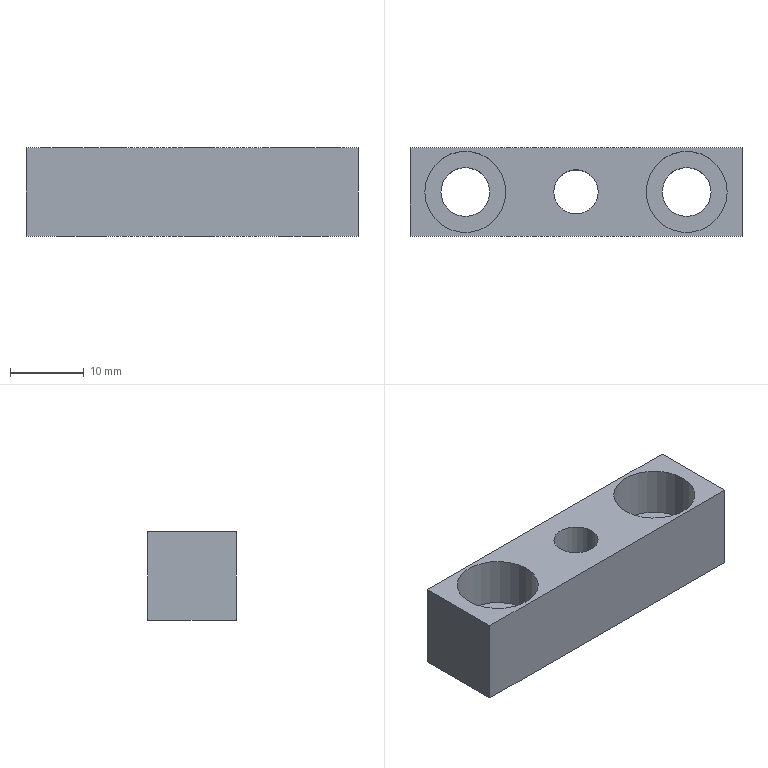Component | NX | GUIDE_BLOCK | 1 solid | 13 faces | box 45 x 12 x 12 mm | volume 4492 mm3 | plane 8 | cylinder 5 | commonest cylinder face diameters 6.6 x2 11 x2 6 x1
STEP:
#1=CARTESIAN_POINT('',(0.,0.,0.));
#2=DIRECTION('',(0.,0.,1.));
#3=DIRECTION('',(1.,0.,0.));
#4=AXIS2_PLACEMENT_3D('',#1,#2,#3);
#5=CARTESIAN_POINT('',(-95.,33.,10.));
#6=VERTEX_POINT('',#5);
#7=CARTESIAN_POINT('',(-95.,21.,10.));
#8=VERTEX_POINT('',#7);
#9=CARTESIAN_POINT('',(-95.,33.,10.));
#10=DIRECTION('',(0.,-1.,0.));
#11=VECTOR('',#10,1.);
#12=LINE('',#9,#11);
#13=CARTESIAN_POINT('',(-95.,33.,22.));
#14=DIRECTION('',(1.,0.,0.));
#15=DIRECTION('',(0.,0.,-1.));
#16=AXIS2_PLACEMENT_3D('',#13,#14,#15);
#17=PLANE('',#16);
#18=CARTESIAN_POINT('',(12.,0.));
#19=DIRECTION('',(0.,-1.));
#20=VECTOR('',#19,1.);
#21=LINE('',#18,#20);
#22=(GEOMETRIC_REPRESENTATION_CONTEXT(2)PARAMETRIC_REPRESENTATION_CONTEXT()REPRESENTATION_CONTEXT('',''));
#23=DEFINITIONAL_REPRESENTATION('',(#21),#22);
#24=PCURVE('',#17,#23);
#25=CARTESIAN_POINT('',(-72.5,27.,10.));
#26=DIRECTION('',(0.,0.,1.));
#27=DIRECTION('',(1.,0.,0.));
#28=AXIS2_PLACEMENT_3D('',#25,#26,#27);
#29=PLANE('',#28);
#30=CARTESIAN_POINT('',(-22.5,6.));
#31=DIRECTION('',(0.,-1.));
#32=VECTOR('',#31,1.);
#33=LINE('',#30,#32);
#34=(GEOMETRIC_REPRESENTATION_CONTEXT(2)PARAMETRIC_REPRESENTATION_CONTEXT()REPRESENTATION_CONTEXT('',''));
#35=DEFINITIONAL_REPRESENTATION('',(#33),#34);
#36=PCURVE('',#29,#35);
#37=SURFACE_CURVE('',#12,(#24,#36),.PCURVE_S1.);
#38=EDGE_CURVE('',#6,#8,#37,.T.);
#39=ORIENTED_EDGE('',*,*,#38,.T.);
#40=CARTESIAN_POINT('',(-95.,21.,22.));
#41=VERTEX_POINT('',#40);
#42=CARTESIAN_POINT('',(-95.,21.,22.));
#43=DIRECTION('',(0.,0.,-1.));
#44=VECTOR('',#43,1.);
#45=LINE('',#42,#44);
#46=CARTESIAN_POINT('',(0.,-12.));
#47=DIRECTION('',(1.,0.));
#48=VECTOR('',#47,1.);
#49=LINE('',#46,#48);
#50=(GEOMETRIC_REPRESENTATION_CONTEXT(2)PARAMETRIC_REPRESENTATION_CONTEXT()REPRESENTATION_CONTEXT('',''));
#51=DEFINITIONAL_REPRESENTATION('',(#49),#50);
#52=PCURVE('',#17,#51);
#53=CARTESIAN_POINT('',(-95.,21.,22.));
#54=DIRECTION('',(0.,1.,0.));
#55=DIRECTION('',(0.,0.,1.));
#56=AXIS2_PLACEMENT_3D('',#53,#54,#55);
#57=PLANE('',#56);
#58=CARTESIAN_POINT('',(0.,0.));
#59=DIRECTION('',(-1.,0.));
#60=VECTOR('',#59,1.);
#61=LINE('',#58,#60);
#62=(GEOMETRIC_REPRESENTATION_CONTEXT(2)PARAMETRIC_REPRESENTATION_CONTEXT()REPRESENTATION_CONTEXT('',''));
#63=DEFINITIONAL_REPRESENTATION('',(#61),#62);
#64=PCURVE('',#57,#63);
#65=SURFACE_CURVE('',#45,(#52,#64),.PCURVE_S1.);
#66=EDGE_CURVE('',#41,#8,#65,.T.);
#67=ORIENTED_EDGE('',*,*,#66,.F.);
#68=CARTESIAN_POINT('',(-95.,33.,22.));
#69=VERTEX_POINT('',#68);
#70=CARTESIAN_POINT('',(-95.,33.,22.));
#71=DIRECTION('',(0.,-1.,0.));
#72=VECTOR('',#71,1.);
#73=LINE('',#70,#72);
#74=CARTESIAN_POINT('',(0.,0.));
#75=DIRECTION('',(0.,-1.));
#76=VECTOR('',#75,1.);
#77=LINE('',#74,#76);
#78=(GEOMETRIC_REPRESENTATION_CONTEXT(2)PARAMETRIC_REPRESENTATION_CONTEXT()REPRESENTATION_CONTEXT('',''));
#79=DEFINITIONAL_REPRESENTATION('',(#77),#78);
#80=PCURVE('',#17,#79);
#81=CARTESIAN_POINT('',(-72.5,27.,22.));
#82=DIRECTION('',(0.,0.,1.));
#83=DIRECTION('',(1.,0.,0.));
#84=AXIS2_PLACEMENT_3D('',#81,#82,#83);
#85=PLANE('',#84);
#86=CARTESIAN_POINT('',(-22.5,6.));
#87=DIRECTION('',(0.,-1.));
#88=VECTOR('',#87,1.);
#89=LINE('',#86,#88);
#90=(GEOMETRIC_REPRESENTATION_CONTEXT(2)PARAMETRIC_REPRESENTATION_CONTEXT()REPRESENTATION_CONTEXT('',''));
#91=DEFINITIONAL_REPRESENTATION('',(#89),#90);
#92=PCURVE('',#85,#91);
#93=SURFACE_CURVE('',#73,(#80,#92),.PCURVE_S1.);
#94=EDGE_CURVE('',#69,#41,#93,.T.);
#95=ORIENTED_EDGE('',*,*,#94,.F.);
#96=CARTESIAN_POINT('',(-95.,33.,22.));
#97=DIRECTION('',(0.,0.,-1.));
#98=VECTOR('',#97,1.);
#99=LINE('',#96,#98);
#100=CARTESIAN_POINT('',(0.,0.));
#101=DIRECTION('',(1.,0.));
#102=VECTOR('',#101,1.);
#103=LINE('',#100,#102);
#104=(GEOMETRIC_REPRESENTATION_CONTEXT(2)PARAMETRIC_REPRESENTATION_CONTEXT()REPRESENTATION_CONTEXT('',''));
#105=DEFINITIONAL_REPRESENTATION('',(#103),#104);
#106=PCURVE('',#17,#105);
#107=CARTESIAN_POINT('',(-50.,33.,22.));
#108=DIRECTION('',(0.,-1.,0.));
#109=DIRECTION('',(0.,0.,-1.));
#110=AXIS2_PLACEMENT_3D('',#107,#108,#109);
#111=PLANE('',#110);
#112=CARTESIAN_POINT('',(0.,-45.));
#113=DIRECTION('',(1.,0.));
#114=VECTOR('',#113,1.);
#115=LINE('',#112,#114);
#116=(GEOMETRIC_REPRESENTATION_CONTEXT(2)PARAMETRIC_REPRESENTATION_CONTEXT()REPRESENTATION_CONTEXT('',''));
#117=DEFINITIONAL_REPRESENTATION('',(#115),#116);
#118=PCURVE('',#111,#117);
#119=SURFACE_CURVE('',#99,(#106,#118),.PCURVE_S1.);
#120=EDGE_CURVE('',#69,#6,#119,.T.);
#121=ORIENTED_EDGE('',*,*,#120,.T.);
#122=EDGE_LOOP('',(#39,#67,#95,#121));
#123=FACE_BOUND('',#122,.T.);
#124=ADVANCED_FACE('',(#123),#17,.F.);
#125=CARTESIAN_POINT('',(-50.,21.,10.));
#126=VERTEX_POINT('',#125);
#127=CARTESIAN_POINT('',(-95.,21.,10.));
#128=DIRECTION('',(1.,0.,0.));
#129=VECTOR('',#128,1.);
#130=LINE('',#127,#129);
#131=CARTESIAN_POINT('',(-12.,0.));
#132=DIRECTION('',(0.,1.));
#133=VECTOR('',#132,1.);
#134=LINE('',#131,#133);
#135=(GEOMETRIC_REPRESENTATION_CONTEXT(2)PARAMETRIC_REPRESENTATION_CONTEXT()REPRESENTATION_CONTEXT('',''));
#136=DEFINITIONAL_REPRESENTATION('',(#134),#135);
#137=PCURVE('',#57,#136);
#138=CARTESIAN_POINT('',(-22.5,-6.));
#139=DIRECTION('',(1.,0.));
#140=VECTOR('',#139,1.);
#141=LINE('',#138,#140);
#142=(GEOMETRIC_REPRESENTATION_CONTEXT(2)PARAMETRIC_REPRESENTATION_CONTEXT()REPRESENTATION_CONTEXT('',''));
#143=DEFINITIONAL_REPRESENTATION('',(#141),#142);
#144=PCURVE('',#29,#143);
#145=SURFACE_CURVE('',#130,(#137,#144),.PCURVE_S1.);
#146=EDGE_CURVE('',#8,#126,#145,.T.);
#147=ORIENTED_EDGE('',*,*,#146,.T.);
#148=CARTESIAN_POINT('',(-50.,21.,22.));
#149=VERTEX_POINT('',#148);
#150=CARTESIAN_POINT('',(-50.,21.,22.));
#151=DIRECTION('',(0.,0.,-1.));
#152=VECTOR('',#151,1.);
#153=LINE('',#150,#152);
#154=CARTESIAN_POINT('',(0.,45.));
#155=DIRECTION('',(-1.,0.));
#156=VECTOR('',#155,1.);
#157=LINE('',#154,#156);
#158=(GEOMETRIC_REPRESENTATION_CONTEXT(2)PARAMETRIC_REPRESENTATION_CONTEXT()REPRESENTATION_CONTEXT('',''));
#159=DEFINITIONAL_REPRESENTATION('',(#157),#158);
#160=PCURVE('',#57,#159);
#161=CARTESIAN_POINT('',(-50.,21.,22.));
#162=DIRECTION('',(-1.,0.,0.));
#163=DIRECTION('',(0.,0.,1.));
#164=AXIS2_PLACEMENT_3D('',#161,#162,#163);
#165=PLANE('',#164);
#166=CARTESIAN_POINT('',(0.,0.));
#167=DIRECTION('',(-1.,0.));
#168=VECTOR('',#167,1.);
#169=LINE('',#166,#168);
#170=(GEOMETRIC_REPRESENTATION_CONTEXT(2)PARAMETRIC_REPRESENTATION_CONTEXT()REPRESENTATION_CONTEXT('',''));
#171=DEFINITIONAL_REPRESENTATION('',(#169),#170);
#172=PCURVE('',#165,#171);
#173=SURFACE_CURVE('',#153,(#160,#172),.PCURVE_S1.);
#174=EDGE_CURVE('',#149,#126,#173,.T.);
#175=ORIENTED_EDGE('',*,*,#174,.F.);
#176=CARTESIAN_POINT('',(-95.,21.,22.));
#177=DIRECTION('',(1.,0.,0.));
#178=VECTOR('',#177,1.);
#179=LINE('',#176,#178);
#180=CARTESIAN_POINT('',(0.,0.));
#181=DIRECTION('',(0.,1.));
#182=VECTOR('',#181,1.);
#183=LINE('',#180,#182);
#184=(GEOMETRIC_REPRESENTATION_CONTEXT(2)PARAMETRIC_REPRESENTATION_CONTEXT()REPRESENTATION_CONTEXT('',''));
#185=DEFINITIONAL_REPRESENTATION('',(#183),#184);
#186=PCURVE('',#57,#185);
#187=CARTESIAN_POINT('',(-22.5,-6.));
#188=DIRECTION('',(1.,0.));
#189=VECTOR('',#188,1.);
#190=LINE('',#187,#189);
#191=(GEOMETRIC_REPRESENTATION_CONTEXT(2)PARAMETRIC_REPRESENTATION_CONTEXT()REPRESENTATION_CONTEXT('',''));
#192=DEFINITIONAL_REPRESENTATION('',(#190),#191);
#193=PCURVE('',#85,#192);
#194=SURFACE_CURVE('',#179,(#186,#193),.PCURVE_S1.);
#195=EDGE_CURVE('',#41,#149,#194,.T.);
#196=ORIENTED_EDGE('',*,*,#195,.F.);
#197=ORIENTED_EDGE('',*,*,#66,.T.);
#198=EDGE_LOOP('',(#147,#175,#196,#197));
#199=FACE_BOUND('',#198,.T.);
#200=ADVANCED_FACE('',(#199),#57,.F.);
#201=CARTESIAN_POINT('',(-50.,33.,10.));
#202=VERTEX_POINT('',#201);
#203=CARTESIAN_POINT('',(-50.,21.,10.));
#204=DIRECTION('',(0.,1.,0.));
#205=VECTOR('',#204,1.);
#206=LINE('',#203,#205);
#207=CARTESIAN_POINT('',(-12.,0.));
#208=DIRECTION('',(0.,1.));
#209=VECTOR('',#208,1.);
#210=LINE('',#207,#209);
#211=(GEOMETRIC_REPRESENTATION_CONTEXT(2)PARAMETRIC_REPRESENTATION_CONTEXT()REPRESENTATION_CONTEXT('',''));
#212=DEFINITIONAL_REPRESENTATION('',(#210),#211);
#213=PCURVE('',#165,#212);
#214=CARTESIAN_POINT('',(22.5,-6.));
#215=DIRECTION('',(0.,1.));
#216=VECTOR('',#215,1.);
#217=LINE('',#214,#216);
#218=(GEOMETRIC_REPRESENTATION_CONTEXT(2)PARAMETRIC_REPRESENTATION_CONTEXT()REPRESENTATION_CONTEXT('',''));
#219=DEFINITIONAL_REPRESENTATION('',(#217),#218);
#220=PCURVE('',#29,#219);
#221=SURFACE_CURVE('',#206,(#213,#220),.PCURVE_S1.);
#222=EDGE_CURVE('',#126,#202,#221,.T.);
#223=ORIENTED_EDGE('',*,*,#222,.T.);
#224=CARTESIAN_POINT('',(-50.,33.,22.));
#225=VERTEX_POINT('',#224);
#226=CARTESIAN_POINT('',(-50.,33.,22.));
#227=DIRECTION('',(0.,0.,-1.));
#228=VECTOR('',#227,1.);
#229=LINE('',#226,#228);
#230=CARTESIAN_POINT('',(0.,12.));
#231=DIRECTION('',(-1.,0.));
#232=VECTOR('',#231,1.);
#233=LINE('',#230,#232);
#234=(GEOMETRIC_REPRESENTATION_CONTEXT(2)PARAMETRIC_REPRESENTATION_CONTEXT()REPRESENTATION_CONTEXT('',''));
#235=DEFINITIONAL_REPRESENTATION('',(#233),#234);
#236=PCURVE('',#165,#235);
#237=CARTESIAN_POINT('',(0.,0.));
#238=DIRECTION('',(1.,0.));
#239=VECTOR('',#238,1.);
#240=LINE('',#237,#239);
#241=(GEOMETRIC_REPRESENTATION_CONTEXT(2)PARAMETRIC_REPRESENTATION_CONTEXT()REPRESENTATION_CONTEXT('',''));
#242=DEFINITIONAL_REPRESENTATION('',(#240),#241);
#243=PCURVE('',#111,#242);
#244=SURFACE_CURVE('',#229,(#236,#243),.PCURVE_S1.);
#245=EDGE_CURVE('',#225,#202,#244,.T.);
#246=ORIENTED_EDGE('',*,*,#245,.F.);
#247=CARTESIAN_POINT('',(-50.,21.,22.));
#248=DIRECTION('',(0.,1.,0.));
#249=VECTOR('',#248,1.);
#250=LINE('',#247,#249);
#251=CARTESIAN_POINT('',(0.,0.));
#252=DIRECTION('',(0.,1.));
#253=VECTOR('',#252,1.);
#254=LINE('',#251,#253);
#255=(GEOMETRIC_REPRESENTATION_CONTEXT(2)PARAMETRIC_REPRESENTATION_CONTEXT()REPRESENTATION_CONTEXT('',''));
#256=DEFINITIONAL_REPRESENTATION('',(#254),#255);
#257=PCURVE('',#165,#256);
#258=CARTESIAN_POINT('',(22.5,-6.));
#259=DIRECTION('',(0.,1.));
#260=VECTOR('',#259,1.);
#261=LINE('',#258,#260);
#262=(GEOMETRIC_REPRESENTATION_CONTEXT(2)PARAMETRIC_REPRESENTATION_CONTEXT()REPRESENTATION_CONTEXT('',''));
#263=DEFINITIONAL_REPRESENTATION('',(#261),#262);
#264=PCURVE('',#85,#263);
#265=SURFACE_CURVE('',#250,(#257,#264),.PCURVE_S1.);
#266=EDGE_CURVE('',#149,#225,#265,.T.);
#267=ORIENTED_EDGE('',*,*,#266,.F.);
#268=ORIENTED_EDGE('',*,*,#174,.T.);
#269=EDGE_LOOP('',(#223,#246,#267,#268));
#270=FACE_BOUND('',#269,.T.);
#271=ADVANCED_FACE('',(#270),#165,.F.);
#272=CARTESIAN_POINT('',(-50.,33.,10.));
#273=DIRECTION('',(-1.,0.,0.));
#274=VECTOR('',#273,1.);
#275=LINE('',#272,#274);
#276=CARTESIAN_POINT('',(12.,0.));
#277=DIRECTION('',(0.,-1.));
#278=VECTOR('',#277,1.);
#279=LINE('',#276,#278);
#280=(GEOMETRIC_REPRESENTATION_CONTEXT(2)PARAMETRIC_REPRESENTATION_CONTEXT()REPRESENTATION_CONTEXT('',''));
#281=DEFINITIONAL_REPRESENTATION('',(#279),#280);
#282=PCURVE('',#111,#281);
#283=CARTESIAN_POINT('',(22.5,6.));
#284=DIRECTION('',(-1.,0.));
#285=VECTOR('',#284,1.);
#286=LINE('',#283,#285);
#287=(GEOMETRIC_REPRESENTATION_CONTEXT(2)PARAMETRIC_REPRESENTATION_CONTEXT()REPRESENTATION_CONTEXT('',''));
#288=DEFINITIONAL_REPRESENTATION('',(#286),#287);
#289=PCURVE('',#29,#288);
#290=SURFACE_CURVE('',#275,(#282,#289),.PCURVE_S1.);
#291=EDGE_CURVE('',#202,#6,#290,.T.);
#292=ORIENTED_EDGE('',*,*,#291,.T.);
#293=ORIENTED_EDGE('',*,*,#120,.F.);
#294=CARTESIAN_POINT('',(-50.,33.,22.));
#295=DIRECTION('',(-1.,0.,0.));
#296=VECTOR('',#295,1.);
#297=LINE('',#294,#296);
#298=CARTESIAN_POINT('',(0.,0.));
#299=DIRECTION('',(0.,-1.));
#300=VECTOR('',#299,1.);
#301=LINE('',#298,#300);
#302=(GEOMETRIC_REPRESENTATION_CONTEXT(2)PARAMETRIC_REPRESENTATION_CONTEXT()REPRESENTATION_CONTEXT('',''));
#303=DEFINITIONAL_REPRESENTATION('',(#301),#302);
#304=PCURVE('',#111,#303);
#305=CARTESIAN_POINT('',(22.5,6.));
#306=DIRECTION('',(-1.,0.));
#307=VECTOR('',#306,1.);
#308=LINE('',#305,#307);
#309=(GEOMETRIC_REPRESENTATION_CONTEXT(2)PARAMETRIC_REPRESENTATION_CONTEXT()REPRESENTATION_CONTEXT('',''));
#310=DEFINITIONAL_REPRESENTATION('',(#308),#309);
#311=PCURVE('',#85,#310);
#312=SURFACE_CURVE('',#297,(#304,#311),.PCURVE_S1.);
#313=EDGE_CURVE('',#225,#69,#312,.T.);
#314=ORIENTED_EDGE('',*,*,#313,.F.);
#315=ORIENTED_EDGE('',*,*,#245,.T.);
#316=EDGE_LOOP('',(#292,#293,#314,#315));
#317=FACE_BOUND('',#316,.T.);
#318=ADVANCED_FACE('',(#317),#111,.F.);
#319=CARTESIAN_POINT('',(-63.,27.,22.));
#320=VERTEX_POINT('',#319);
#321=CARTESIAN_POINT('',(-57.5,27.,22.));
#322=DIRECTION('',(0.,0.,-1.));
#323=DIRECTION('',(-1.,0.,0.));
#324=AXIS2_PLACEMENT_3D('',#321,#322,#323);
#325=CIRCLE('',#324,5.5);
#326=CARTESIAN_POINT('',(9.5,0.));
#327=CARTESIAN_POINT('',(9.5,9.526));
#328=CARTESIAN_POINT('',(17.75,4.763));
#329=CARTESIAN_POINT('',(26.,0.));
#330=CARTESIAN_POINT('',(17.75,-4.763));
#331=CARTESIAN_POINT('',(9.5,-9.526));
#332=CARTESIAN_POINT('',(9.5,0.));
#333=(BOUNDED_CURVE()B_SPLINE_CURVE(2,(#326,#327,#328,#329,#330,#331,#332),.UNSPECIFIED.,.T.,.F.)B_SPLINE_CURVE_WITH_KNOTS((1,2,2,2,2,1),(-2.094,0.,2.094,4.189,6.283,8.378),.UNSPECIFIED.)CURVE()GEOMETRIC_REPRESENTATION_ITEM()RATIONAL_B_SPLINE_CURVE((1.,0.5,1.,0.5,1.,0.5,1.))REPRESENTATION_ITEM(''));
#334=(GEOMETRIC_REPRESENTATION_CONTEXT(2)PARAMETRIC_REPRESENTATION_CONTEXT()REPRESENTATION_CONTEXT('',''));
#335=DEFINITIONAL_REPRESENTATION('',(#333),#334);
#336=PCURVE('',#85,#335);
#337=CARTESIAN_POINT('',(-57.5,27.,22.));
#338=DIRECTION('',(0.,0.,-1.));
#339=DIRECTION('',(-1.,0.,0.));
#340=AXIS2_PLACEMENT_3D('',#337,#338,#339);
#341=CYLINDRICAL_SURFACE('',#340,5.5);
#342=CARTESIAN_POINT('',(0.,0.));
#343=DIRECTION('',(1.,0.));
#344=VECTOR('',#343,1.);
#345=LINE('',#342,#344);
#346=(GEOMETRIC_REPRESENTATION_CONTEXT(2)PARAMETRIC_REPRESENTATION_CONTEXT()REPRESENTATION_CONTEXT('',''));
#347=DEFINITIONAL_REPRESENTATION('',(#345),#346);
#348=PCURVE('',#341,#347);
#349=SURFACE_CURVE('',#325,(#336,#348),.PCURVE_S1.);
#350=EDGE_CURVE('',#320,#320,#349,.T.);
#351=ORIENTED_EDGE('',*,*,#350,.T.);
#352=EDGE_LOOP('',(#351));
#353=FACE_BOUND('',#352,.T.);
#354=CARTESIAN_POINT('',(-93.,27.,22.));
#355=VERTEX_POINT('',#354);
#356=CARTESIAN_POINT('',(-87.5,27.,22.));
#357=DIRECTION('',(0.,0.,-1.));
#358=DIRECTION('',(-1.,0.,0.));
#359=AXIS2_PLACEMENT_3D('',#356,#357,#358);
#360=CIRCLE('',#359,5.5);
#361=CARTESIAN_POINT('',(-20.5,0.));
#362=CARTESIAN_POINT('',(-20.5,9.526));
#363=CARTESIAN_POINT('',(-12.25,4.763));
#364=CARTESIAN_POINT('',(-4.,0.));
#365=CARTESIAN_POINT('',(-12.25,-4.763));
#366=CARTESIAN_POINT('',(-20.5,-9.526));
#367=CARTESIAN_POINT('',(-20.5,0.));
#368=(BOUNDED_CURVE()B_SPLINE_CURVE(2,(#361,#362,#363,#364,#365,#366,#367),.UNSPECIFIED.,.T.,.F.)B_SPLINE_CURVE_WITH_KNOTS((1,2,2,2,2,1),(-2.094,0.,2.094,4.189,6.283,8.378),.UNSPECIFIED.)CURVE()GEOMETRIC_REPRESENTATION_ITEM()RATIONAL_B_SPLINE_CURVE((1.,0.5,1.,0.5,1.,0.5,1.))REPRESENTATION_ITEM(''));
#369=(GEOMETRIC_REPRESENTATION_CONTEXT(2)PARAMETRIC_REPRESENTATION_CONTEXT()REPRESENTATION_CONTEXT('',''));
#370=DEFINITIONAL_REPRESENTATION('',(#368),#369);
#371=PCURVE('',#85,#370);
#372=CARTESIAN_POINT('',(-87.5,27.,22.));
#373=DIRECTION('',(0.,0.,-1.));
#374=DIRECTION('',(-1.,0.,0.));
#375=AXIS2_PLACEMENT_3D('',#372,#373,#374);
#376=CYLINDRICAL_SURFACE('',#375,5.5);
#377=CARTESIAN_POINT('',(0.,0.));
#378=DIRECTION('',(1.,0.));
#379=VECTOR('',#378,1.);
#380=LINE('',#377,#379);
#381=(GEOMETRIC_REPRESENTATION_CONTEXT(2)PARAMETRIC_REPRESENTATION_CONTEXT()REPRESENTATION_CONTEXT('',''));
#382=DEFINITIONAL_REPRESENTATION('',(#380),#381);
#383=PCURVE('',#376,#382);
#384=SURFACE_CURVE('',#360,(#371,#383),.PCURVE_S1.);
#385=EDGE_CURVE('',#355,#355,#384,.T.);
#386=ORIENTED_EDGE('',*,*,#385,.T.);
#387=EDGE_LOOP('',(#386));
#388=FACE_BOUND('',#387,.T.);
#389=CARTESIAN_POINT('',(-75.5,27.,22.));
#390=VERTEX_POINT('',#389);
#391=CARTESIAN_POINT('',(-72.5,27.,22.));
#392=DIRECTION('',(0.,0.,-1.));
#393=DIRECTION('',(-1.,0.,0.));
#394=AXIS2_PLACEMENT_3D('',#391,#392,#393);
#395=CIRCLE('',#394,3.);
#396=CARTESIAN_POINT('',(-3.,0.));
#397=CARTESIAN_POINT('',(-3.,5.196));
#398=CARTESIAN_POINT('',(1.5,2.598));
#399=CARTESIAN_POINT('',(6.,0.));
#400=CARTESIAN_POINT('',(1.5,-2.598));
#401=CARTESIAN_POINT('',(-3.,-5.196));
#402=CARTESIAN_POINT('',(-3.,0.));
#403=(BOUNDED_CURVE()B_SPLINE_CURVE(2,(#396,#397,#398,#399,#400,#401,#402),.UNSPECIFIED.,.T.,.F.)B_SPLINE_CURVE_WITH_KNOTS((1,2,2,2,2,1),(-2.094,0.,2.094,4.189,6.283,8.378),.UNSPECIFIED.)CURVE()GEOMETRIC_REPRESENTATION_ITEM()RATIONAL_B_SPLINE_CURVE((1.,0.5,1.,0.5,1.,0.5,1.))REPRESENTATION_ITEM(''));
#404=(GEOMETRIC_REPRESENTATION_CONTEXT(2)PARAMETRIC_REPRESENTATION_CONTEXT()REPRESENTATION_CONTEXT('',''));
#405=DEFINITIONAL_REPRESENTATION('',(#403),#404);
#406=PCURVE('',#85,#405);
#407=CARTESIAN_POINT('',(-72.5,27.,22.));
#408=DIRECTION('',(0.,0.,-1.));
#409=DIRECTION('',(-1.,0.,0.));
#410=AXIS2_PLACEMENT_3D('',#407,#408,#409);
#411=CYLINDRICAL_SURFACE('',#410,3.);
#412=CARTESIAN_POINT('',(0.,0.));
#413=DIRECTION('',(1.,0.));
#414=VECTOR('',#413,1.);
#415=LINE('',#412,#414);
#416=(GEOMETRIC_REPRESENTATION_CONTEXT(2)PARAMETRIC_REPRESENTATION_CONTEXT()REPRESENTATION_CONTEXT('',''));
#417=DEFINITIONAL_REPRESENTATION('',(#415),#416);
#418=PCURVE('',#411,#417);
#419=SURFACE_CURVE('',#395,(#406,#418),.PCURVE_S1.);
#420=EDGE_CURVE('',#390,#390,#419,.T.);
#421=ORIENTED_EDGE('',*,*,#420,.T.);
#422=EDGE_LOOP('',(#421));
#423=FACE_BOUND('',#422,.T.);
#424=ORIENTED_EDGE('',*,*,#94,.T.);
#425=ORIENTED_EDGE('',*,*,#195,.T.);
#426=ORIENTED_EDGE('',*,*,#266,.T.);
#427=ORIENTED_EDGE('',*,*,#313,.T.);
#428=EDGE_LOOP('',(#424,#425,#426,#427));
#429=FACE_BOUND('',#428,.T.);
#430=ADVANCED_FACE('',(#353,#388,#423,#429),#85,.T.);
#431=CARTESIAN_POINT('',(-54.2,27.,10.));
#432=VERTEX_POINT('',#431);
#433=CARTESIAN_POINT('',(-60.8,27.,10.));
#434=VERTEX_POINT('',#433);
#435=CARTESIAN_POINT('',(-57.5,27.,10.));
#436=DIRECTION('',(0.,0.,1.));
#437=DIRECTION('',(1.,0.,0.));
#438=AXIS2_PLACEMENT_3D('',#435,#436,#437);
#439=CIRCLE('',#438,3.3);
#440=CARTESIAN_POINT('',(15.,0.));
#441=DIRECTION('',(1.,0.));
#442=AXIS2_PLACEMENT_2D('',#440,#441);
#443=CIRCLE('',#442,3.3);
#444=(GEOMETRIC_REPRESENTATION_CONTEXT(2)PARAMETRIC_REPRESENTATION_CONTEXT()REPRESENTATION_CONTEXT('',''));
#445=DEFINITIONAL_REPRESENTATION('',(#443),#444);
#446=PCURVE('',#29,#445);
#447=CARTESIAN_POINT('',(-57.5,27.,-5.787));
#448=DIRECTION('',(0.,0.,-1.));
#449=DIRECTION('',(-1.,0.,0.));
#450=AXIS2_PLACEMENT_3D('',#447,#448,#449);
#451=CYLINDRICAL_SURFACE('',#450,3.3);
#452=CARTESIAN_POINT('',(3.142,-15.787));
#453=DIRECTION('',(-1.,0.));
#454=VECTOR('',#453,1.);
#455=LINE('',#452,#454);
#456=(GEOMETRIC_REPRESENTATION_CONTEXT(2)PARAMETRIC_REPRESENTATION_CONTEXT()REPRESENTATION_CONTEXT('',''));
#457=DEFINITIONAL_REPRESENTATION('',(#455),#456);
#458=PCURVE('',#451,#457);
#459=SURFACE_CURVE('',#439,(#446,#458),.PCURVE_S1.);
#460=EDGE_CURVE('',#432,#434,#459,.T.);
#461=ORIENTED_EDGE('',*,*,#460,.T.);
#462=CARTESIAN_POINT('',(-57.5,27.,10.));
#463=DIRECTION('',(0.,0.,1.));
#464=DIRECTION('',(1.,0.,0.));
#465=AXIS2_PLACEMENT_3D('',#462,#463,#464);
#466=CIRCLE('',#465,3.3);
#467=CARTESIAN_POINT('',(15.,0.));
#468=DIRECTION('',(1.,0.));
#469=AXIS2_PLACEMENT_2D('',#467,#468);
#470=CIRCLE('',#469,3.3);
#471=(GEOMETRIC_REPRESENTATION_CONTEXT(2)PARAMETRIC_REPRESENTATION_CONTEXT()REPRESENTATION_CONTEXT('',''));
#472=DEFINITIONAL_REPRESENTATION('',(#470),#471);
#473=PCURVE('',#29,#472);
#474=CARTESIAN_POINT('',(9.425,-15.787));
#475=DIRECTION('',(-1.,0.));
#476=VECTOR('',#475,1.);
#477=LINE('',#474,#476);
#478=(GEOMETRIC_REPRESENTATION_CONTEXT(2)PARAMETRIC_REPRESENTATION_CONTEXT()REPRESENTATION_CONTEXT('',''));
#479=DEFINITIONAL_REPRESENTATION('',(#477),#478);
#480=PCURVE('',#451,#479);
#481=SURFACE_CURVE('',#466,(#473,#480),.PCURVE_S1.);
#482=EDGE_CURVE('',#434,#432,#481,.T.);
#483=ORIENTED_EDGE('',*,*,#482,.T.);
#484=EDGE_LOOP('',(#461,#483));
#485=FACE_BOUND('',#484,.T.);
#486=CARTESIAN_POINT('',(-84.2,27.,10.));
#487=VERTEX_POINT('',#486);
#488=CARTESIAN_POINT('',(-90.8,27.,10.));
#489=VERTEX_POINT('',#488);
#490=CARTESIAN_POINT('',(-87.5,27.,10.));
#491=DIRECTION('',(0.,0.,1.));
#492=DIRECTION('',(1.,0.,0.));
#493=AXIS2_PLACEMENT_3D('',#490,#491,#492);
#494=CIRCLE('',#493,3.3);
#495=CARTESIAN_POINT('',(-15.,0.));
#496=DIRECTION('',(1.,0.));
#497=AXIS2_PLACEMENT_2D('',#495,#496);
#498=CIRCLE('',#497,3.3);
#499=(GEOMETRIC_REPRESENTATION_CONTEXT(2)PARAMETRIC_REPRESENTATION_CONTEXT()REPRESENTATION_CONTEXT('',''));
#500=DEFINITIONAL_REPRESENTATION('',(#498),#499);
#501=PCURVE('',#29,#500);
#502=CARTESIAN_POINT('',(-87.5,27.,-5.787));
#503=DIRECTION('',(0.,0.,-1.));
#504=DIRECTION('',(-1.,0.,0.));
#505=AXIS2_PLACEMENT_3D('',#502,#503,#504);
#506=CYLINDRICAL_SURFACE('',#505,3.3);
#507=CARTESIAN_POINT('',(3.142,-15.787));
#508=DIRECTION('',(-1.,0.));
#509=VECTOR('',#508,1.);
#510=LINE('',#507,#509);
#511=(GEOMETRIC_REPRESENTATION_CONTEXT(2)PARAMETRIC_REPRESENTATION_CONTEXT()REPRESENTATION_CONTEXT('',''));
#512=DEFINITIONAL_REPRESENTATION('',(#510),#511);
#513=PCURVE('',#506,#512);
#514=SURFACE_CURVE('',#494,(#501,#513),.PCURVE_S1.);
#515=EDGE_CURVE('',#487,#489,#514,.T.);
#516=ORIENTED_EDGE('',*,*,#515,.T.);
#517=CARTESIAN_POINT('',(-87.5,27.,10.));
#518=DIRECTION('',(0.,0.,1.));
#519=DIRECTION('',(1.,0.,0.));
#520=AXIS2_PLACEMENT_3D('',#517,#518,#519);
#521=CIRCLE('',#520,3.3);
#522=CARTESIAN_POINT('',(-15.,0.));
#523=DIRECTION('',(1.,0.));
#524=AXIS2_PLACEMENT_2D('',#522,#523);
#525=CIRCLE('',#524,3.3);
#526=(GEOMETRIC_REPRESENTATION_CONTEXT(2)PARAMETRIC_REPRESENTATION_CONTEXT()REPRESENTATION_CONTEXT('',''));
#527=DEFINITIONAL_REPRESENTATION('',(#525),#526);
#528=PCURVE('',#29,#527);
#529=CARTESIAN_POINT('',(9.425,-15.787));
#530=DIRECTION('',(-1.,0.));
#531=VECTOR('',#530,1.);
#532=LINE('',#529,#531);
#533=(GEOMETRIC_REPRESENTATION_CONTEXT(2)PARAMETRIC_REPRESENTATION_CONTEXT()REPRESENTATION_CONTEXT('',''));
#534=DEFINITIONAL_REPRESENTATION('',(#532),#533);
#535=PCURVE('',#506,#534);
#536=SURFACE_CURVE('',#521,(#528,#535),.PCURVE_S1.);
#537=EDGE_CURVE('',#489,#487,#536,.T.);
#538=ORIENTED_EDGE('',*,*,#537,.T.);
#539=EDGE_LOOP('',(#516,#538));
#540=FACE_BOUND('',#539,.T.);
#541=CARTESIAN_POINT('',(-69.5,27.,10.));
#542=VERTEX_POINT('',#541);
#543=CARTESIAN_POINT('',(-75.5,27.,10.));
#544=VERTEX_POINT('',#543);
#545=CARTESIAN_POINT('',(-72.5,27.,10.));
#546=DIRECTION('',(0.,0.,1.));
#547=DIRECTION('',(1.,0.,0.));
#548=AXIS2_PLACEMENT_3D('',#545,#546,#547);
#549=CIRCLE('',#548,3.);
#550=CARTESIAN_POINT('',(0.,0.));
#551=DIRECTION('',(1.,0.));
#552=AXIS2_PLACEMENT_2D('',#550,#551);
#553=CIRCLE('',#552,3.);
#554=(GEOMETRIC_REPRESENTATION_CONTEXT(2)PARAMETRIC_REPRESENTATION_CONTEXT()REPRESENTATION_CONTEXT('',''));
#555=DEFINITIONAL_REPRESENTATION('',(#553),#554);
#556=PCURVE('',#29,#555);
#557=CARTESIAN_POINT('',(3.142,12.));
#558=DIRECTION('',(-1.,0.));
#559=VECTOR('',#558,1.);
#560=LINE('',#557,#559);
#561=(GEOMETRIC_REPRESENTATION_CONTEXT(2)PARAMETRIC_REPRESENTATION_CONTEXT()REPRESENTATION_CONTEXT('',''));
#562=DEFINITIONAL_REPRESENTATION('',(#560),#561);
#563=PCURVE('',#411,#562);
#564=SURFACE_CURVE('',#549,(#556,#563),.PCURVE_S1.);
#565=EDGE_CURVE('',#542,#544,#564,.T.);
#566=ORIENTED_EDGE('',*,*,#565,.T.);
#567=CARTESIAN_POINT('',(-72.5,27.,10.));
#568=DIRECTION('',(0.,0.,1.));
#569=DIRECTION('',(1.,0.,0.));
#570=AXIS2_PLACEMENT_3D('',#567,#568,#569);
#571=CIRCLE('',#570,3.);
#572=CARTESIAN_POINT('',(0.,0.));
#573=DIRECTION('',(1.,0.));
#574=AXIS2_PLACEMENT_2D('',#572,#573);
#575=CIRCLE('',#574,3.);
#576=(GEOMETRIC_REPRESENTATION_CONTEXT(2)PARAMETRIC_REPRESENTATION_CONTEXT()REPRESENTATION_CONTEXT('',''));
#577=DEFINITIONAL_REPRESENTATION('',(#575),#576);
#578=PCURVE('',#29,#577);
#579=CARTESIAN_POINT('',(9.425,12.));
#580=DIRECTION('',(-1.,0.));
#581=VECTOR('',#580,1.);
#582=LINE('',#579,#581);
#583=(GEOMETRIC_REPRESENTATION_CONTEXT(2)PARAMETRIC_REPRESENTATION_CONTEXT()REPRESENTATION_CONTEXT('',''));
#584=DEFINITIONAL_REPRESENTATION('',(#582),#583);
#585=PCURVE('',#411,#584);
#586=SURFACE_CURVE('',#571,(#578,#585),.PCURVE_S1.);
#587=EDGE_CURVE('',#544,#542,#586,.T.);
#588=ORIENTED_EDGE('',*,*,#587,.T.);
#589=EDGE_LOOP('',(#566,#588));
#590=FACE_BOUND('',#589,.T.);
#591=ORIENTED_EDGE('',*,*,#38,.F.);
#592=ORIENTED_EDGE('',*,*,#291,.F.);
#593=ORIENTED_EDGE('',*,*,#222,.F.);
#594=ORIENTED_EDGE('',*,*,#146,.F.);
#595=EDGE_LOOP('',(#591,#592,#593,#594));
#596=FACE_BOUND('',#595,.T.);
#597=ADVANCED_FACE('',(#485,#540,#590,#596),#29,.F.);
#598=ORIENTED_EDGE('',*,*,#420,.T.);
#599=CARTESIAN_POINT('',(-75.5,27.,22.));
#600=CARTESIAN_POINT('',(-75.5,27.,10.));
#601=B_SPLINE_CURVE_WITH_KNOTS('',1,(#599,#600),.UNSPECIFIED.,.F.,.F.,(2,2),(0.,12.),.PIECEWISE_BEZIER_KNOTS.);
#602=CARTESIAN_POINT('',(6.283,0.));
#603=DIRECTION('',(0.,1.));
#604=VECTOR('',#603,1.);
#605=LINE('',#602,#604);
#606=(GEOMETRIC_REPRESENTATION_CONTEXT(2)PARAMETRIC_REPRESENTATION_CONTEXT()REPRESENTATION_CONTEXT('',''));
#607=DEFINITIONAL_REPRESENTATION('',(#605),#606);
#608=PCURVE('',#411,#607);
#609=CARTESIAN_POINT('',(0.,0.));
#610=DIRECTION('',(0.,1.));
#611=VECTOR('',#610,1.);
#612=LINE('',#609,#611);
#613=(GEOMETRIC_REPRESENTATION_CONTEXT(2)PARAMETRIC_REPRESENTATION_CONTEXT()REPRESENTATION_CONTEXT('',''));
#614=DEFINITIONAL_REPRESENTATION('',(#612),#613);
#615=PCURVE('',#411,#614);
#616=SEAM_CURVE('',#601,(#608,#615),.PCURVE_S1.);
#617=EDGE_CURVE('',#390,#544,#616,.T.);
#618=ORIENTED_EDGE('',*,*,#617,.T.);
#619=ORIENTED_EDGE('',*,*,#587,.T.);
#620=ORIENTED_EDGE('',*,*,#565,.T.);
#621=ORIENTED_EDGE('',*,*,#617,.F.);
#622=EDGE_LOOP('',(#598,#618,#619,#620,#621));
#623=FACE_BOUND('',#622,.F.);
#624=ADVANCED_FACE('',(#623),#411,.F.);
#625=CARTESIAN_POINT('',(-90.8,27.,15.2));
#626=VERTEX_POINT('',#625);
#627=CARTESIAN_POINT('',(-87.5,27.,15.2));
#628=DIRECTION('',(0.,0.,1.));
#629=DIRECTION('',(-1.,0.,0.));
#630=AXIS2_PLACEMENT_3D('',#627,#628,#629);
#631=CIRCLE('',#630,3.3);
#632=CARTESIAN_POINT('',(6.283,-20.987));
#633=DIRECTION('',(-1.,0.));
#634=VECTOR('',#633,1.);
#635=LINE('',#632,#634);
#636=(GEOMETRIC_REPRESENTATION_CONTEXT(2)PARAMETRIC_REPRESENTATION_CONTEXT()REPRESENTATION_CONTEXT('',''));
#637=DEFINITIONAL_REPRESENTATION('',(#635),#636);
#638=PCURVE('',#506,#637);
#639=CARTESIAN_POINT('',(-87.5,27.,15.2));
#640=DIRECTION('',(0.,0.,-1.));
#641=DIRECTION('',(-1.,0.,0.));
#642=AXIS2_PLACEMENT_3D('',#639,#640,#641);
#643=PLANE('',#642);
#644=CARTESIAN_POINT('',(3.3,0.));
#645=CARTESIAN_POINT('',(3.3,-5.716));
#646=CARTESIAN_POINT('',(-1.65,-2.858));
#647=CARTESIAN_POINT('',(-6.6,-0.));
#648=CARTESIAN_POINT('',(-1.65,2.858));
#649=CARTESIAN_POINT('',(3.3,5.716));
#650=CARTESIAN_POINT('',(3.3,0.));
#651=(BOUNDED_CURVE()B_SPLINE_CURVE(2,(#644,#645,#646,#647,#648,#649,#650),.UNSPECIFIED.,.T.,.F.)B_SPLINE_CURVE_WITH_KNOTS((1,2,2,2,2,1),(-2.094,0.,2.094,4.189,6.283,8.378),.UNSPECIFIED.)CURVE()GEOMETRIC_REPRESENTATION_ITEM()RATIONAL_B_SPLINE_CURVE((1.,0.5,1.,0.5,1.,0.5,1.))REPRESENTATION_ITEM(''));
#652=(GEOMETRIC_REPRESENTATION_CONTEXT(2)PARAMETRIC_REPRESENTATION_CONTEXT()REPRESENTATION_CONTEXT('',''));
#653=DEFINITIONAL_REPRESENTATION('',(#651),#652);
#654=PCURVE('',#643,#653);
#655=SURFACE_CURVE('',#631,(#638,#654),.PCURVE_S1.);
#656=EDGE_CURVE('',#626,#626,#655,.T.);
#657=ORIENTED_EDGE('',*,*,#656,.F.);
#658=CARTESIAN_POINT('',(-90.8,27.,15.2));
#659=CARTESIAN_POINT('',(-90.8,27.,10.));
#660=B_SPLINE_CURVE_WITH_KNOTS('',1,(#658,#659),.UNSPECIFIED.,.F.,.F.,(2,2),(-20.987,-15.787),.PIECEWISE_BEZIER_KNOTS.);
#661=CARTESIAN_POINT('',(6.283,0.));
#662=DIRECTION('',(0.,1.));
#663=VECTOR('',#662,1.);
#664=LINE('',#661,#663);
#665=(GEOMETRIC_REPRESENTATION_CONTEXT(2)PARAMETRIC_REPRESENTATION_CONTEXT()REPRESENTATION_CONTEXT('',''));
#666=DEFINITIONAL_REPRESENTATION('',(#664),#665);
#667=PCURVE('',#506,#666);
#668=CARTESIAN_POINT('',(0.,0.));
#669=DIRECTION('',(0.,1.));
#670=VECTOR('',#669,1.);
#671=LINE('',#668,#670);
#672=(GEOMETRIC_REPRESENTATION_CONTEXT(2)PARAMETRIC_REPRESENTATION_CONTEXT()REPRESENTATION_CONTEXT('',''));
#673=DEFINITIONAL_REPRESENTATION('',(#671),#672);
#674=PCURVE('',#506,#673);
#675=SEAM_CURVE('',#660,(#667,#674),.PCURVE_S1.);
#676=EDGE_CURVE('',#626,#489,#675,.T.);
#677=ORIENTED_EDGE('',*,*,#676,.T.);
#678=ORIENTED_EDGE('',*,*,#537,.T.);
#679=ORIENTED_EDGE('',*,*,#515,.T.);
#680=ORIENTED_EDGE('',*,*,#676,.F.);
#681=EDGE_LOOP('',(#657,#677,#678,#679,#680));
#682=FACE_BOUND('',#681,.F.);
#683=ADVANCED_FACE('',(#682),#506,.F.);
#684=ORIENTED_EDGE('',*,*,#656,.F.);
#685=EDGE_LOOP('',(#684));
#686=FACE_BOUND('',#685,.T.);
#687=CARTESIAN_POINT('',(-93.,27.,15.2));
#688=VERTEX_POINT('',#687);
#689=CARTESIAN_POINT('',(-87.5,27.,15.2));
#690=DIRECTION('',(0.,0.,1.));
#691=DIRECTION('',(-1.,0.,0.));
#692=AXIS2_PLACEMENT_3D('',#689,#690,#691);
#693=CIRCLE('',#692,5.5);
#694=CARTESIAN_POINT('',(5.5,0.));
#695=CARTESIAN_POINT('',(5.5,-9.526));
#696=CARTESIAN_POINT('',(-2.75,-4.763));
#697=CARTESIAN_POINT('',(-11.,-0.));
#698=CARTESIAN_POINT('',(-2.75,4.763));
#699=CARTESIAN_POINT('',(5.5,9.526));
#700=CARTESIAN_POINT('',(5.5,0.));
#701=(BOUNDED_CURVE()B_SPLINE_CURVE(2,(#694,#695,#696,#697,#698,#699,#700),.UNSPECIFIED.,.T.,.F.)B_SPLINE_CURVE_WITH_KNOTS((1,2,2,2,2,1),(-2.094,0.,2.094,4.189,6.283,8.378),.UNSPECIFIED.)CURVE()GEOMETRIC_REPRESENTATION_ITEM()RATIONAL_B_SPLINE_CURVE((1.,0.5,1.,0.5,1.,0.5,1.))REPRESENTATION_ITEM(''));
#702=(GEOMETRIC_REPRESENTATION_CONTEXT(2)PARAMETRIC_REPRESENTATION_CONTEXT()REPRESENTATION_CONTEXT('',''));
#703=DEFINITIONAL_REPRESENTATION('',(#701),#702);
#704=PCURVE('',#643,#703);
#705=CARTESIAN_POINT('',(6.283,6.8));
#706=DIRECTION('',(-1.,0.));
#707=VECTOR('',#706,1.);
#708=LINE('',#705,#707);
#709=(GEOMETRIC_REPRESENTATION_CONTEXT(2)PARAMETRIC_REPRESENTATION_CONTEXT()REPRESENTATION_CONTEXT('',''));
#710=DEFINITIONAL_REPRESENTATION('',(#708),#709);
#711=PCURVE('',#376,#710);
#712=SURFACE_CURVE('',#693,(#704,#711),.PCURVE_S1.);
#713=EDGE_CURVE('',#688,#688,#712,.T.);
#714=ORIENTED_EDGE('',*,*,#713,.T.);
#715=EDGE_LOOP('',(#714));
#716=FACE_BOUND('',#715,.T.);
#717=ADVANCED_FACE('',(#686,#716),#643,.F.);
#718=ORIENTED_EDGE('',*,*,#713,.T.);
#719=CARTESIAN_POINT('',(-93.,27.,22.));
#720=CARTESIAN_POINT('',(-93.,27.,15.2));
#721=B_SPLINE_CURVE_WITH_KNOTS('',1,(#719,#720),.UNSPECIFIED.,.F.,.F.,(2,2),(0.,6.8),.PIECEWISE_BEZIER_KNOTS.);
#722=CARTESIAN_POINT('',(0.,0.));
#723=DIRECTION('',(0.,1.));
#724=VECTOR('',#723,1.);
#725=LINE('',#722,#724);
#726=(GEOMETRIC_REPRESENTATION_CONTEXT(2)PARAMETRIC_REPRESENTATION_CONTEXT()REPRESENTATION_CONTEXT('',''));
#727=DEFINITIONAL_REPRESENTATION('',(#725),#726);
#728=PCURVE('',#376,#727);
#729=CARTESIAN_POINT('',(6.283,0.));
#730=DIRECTION('',(0.,1.));
#731=VECTOR('',#730,1.);
#732=LINE('',#729,#731);
#733=(GEOMETRIC_REPRESENTATION_CONTEXT(2)PARAMETRIC_REPRESENTATION_CONTEXT()REPRESENTATION_CONTEXT('',''));
#734=DEFINITIONAL_REPRESENTATION('',(#732),#733);
#735=PCURVE('',#376,#734);
#736=SEAM_CURVE('',#721,(#728,#735),.PCURVE_S1.);
#737=EDGE_CURVE('',#355,#688,#736,.T.);
#738=ORIENTED_EDGE('',*,*,#737,.F.);
#739=ORIENTED_EDGE('',*,*,#385,.T.);
#740=ORIENTED_EDGE('',*,*,#737,.T.);
#741=EDGE_LOOP('',(#718,#738,#739,#740));
#742=FACE_BOUND('',#741,.F.);
#743=ADVANCED_FACE('',(#742),#376,.F.);
#744=CARTESIAN_POINT('',(-60.8,27.,15.2));
#745=VERTEX_POINT('',#744);
#746=CARTESIAN_POINT('',(-57.5,27.,15.2));
#747=DIRECTION('',(0.,0.,1.));
#748=DIRECTION('',(-1.,0.,0.));
#749=AXIS2_PLACEMENT_3D('',#746,#747,#748);
#750=CIRCLE('',#749,3.3);
#751=CARTESIAN_POINT('',(6.283,-20.987));
#752=DIRECTION('',(-1.,0.));
#753=VECTOR('',#752,1.);
#754=LINE('',#751,#753);
#755=(GEOMETRIC_REPRESENTATION_CONTEXT(2)PARAMETRIC_REPRESENTATION_CONTEXT()REPRESENTATION_CONTEXT('',''));
#756=DEFINITIONAL_REPRESENTATION('',(#754),#755);
#757=PCURVE('',#451,#756);
#758=CARTESIAN_POINT('',(-57.5,27.,15.2));
#759=DIRECTION('',(0.,0.,-1.));
#760=DIRECTION('',(-1.,0.,0.));
#761=AXIS2_PLACEMENT_3D('',#758,#759,#760);
#762=PLANE('',#761);
#763=CARTESIAN_POINT('',(3.3,0.));
#764=CARTESIAN_POINT('',(3.3,-5.716));
#765=CARTESIAN_POINT('',(-1.65,-2.858));
#766=CARTESIAN_POINT('',(-6.6,-0.));
#767=CARTESIAN_POINT('',(-1.65,2.858));
#768=CARTESIAN_POINT('',(3.3,5.716));
#769=CARTESIAN_POINT('',(3.3,0.));
#770=(BOUNDED_CURVE()B_SPLINE_CURVE(2,(#763,#764,#765,#766,#767,#768,#769),.UNSPECIFIED.,.T.,.F.)B_SPLINE_CURVE_WITH_KNOTS((1,2,2,2,2,1),(-2.094,0.,2.094,4.189,6.283,8.378),.UNSPECIFIED.)CURVE()GEOMETRIC_REPRESENTATION_ITEM()RATIONAL_B_SPLINE_CURVE((1.,0.5,1.,0.5,1.,0.5,1.))REPRESENTATION_ITEM(''));
#771=(GEOMETRIC_REPRESENTATION_CONTEXT(2)PARAMETRIC_REPRESENTATION_CONTEXT()REPRESENTATION_CONTEXT('',''));
#772=DEFINITIONAL_REPRESENTATION('',(#770),#771);
#773=PCURVE('',#762,#772);
#774=SURFACE_CURVE('',#750,(#757,#773),.PCURVE_S1.);
#775=EDGE_CURVE('',#745,#745,#774,.T.);
#776=ORIENTED_EDGE('',*,*,#775,.F.);
#777=CARTESIAN_POINT('',(-60.8,27.,15.2));
#778=CARTESIAN_POINT('',(-60.8,27.,10.));
#779=B_SPLINE_CURVE_WITH_KNOTS('',1,(#777,#778),.UNSPECIFIED.,.F.,.F.,(2,2),(-20.987,-15.787),.PIECEWISE_BEZIER_KNOTS.);
#780=CARTESIAN_POINT('',(6.283,0.));
#781=DIRECTION('',(0.,1.));
#782=VECTOR('',#781,1.);
#783=LINE('',#780,#782);
#784=(GEOMETRIC_REPRESENTATION_CONTEXT(2)PARAMETRIC_REPRESENTATION_CONTEXT()REPRESENTATION_CONTEXT('',''));
#785=DEFINITIONAL_REPRESENTATION('',(#783),#784);
#786=PCURVE('',#451,#785);
#787=CARTESIAN_POINT('',(0.,0.));
#788=DIRECTION('',(0.,1.));
#789=VECTOR('',#788,1.);
#790=LINE('',#787,#789);
#791=(GEOMETRIC_REPRESENTATION_CONTEXT(2)PARAMETRIC_REPRESENTATION_CONTEXT()REPRESENTATION_CONTEXT('',''));
#792=DEFINITIONAL_REPRESENTATION('',(#790),#791);
#793=PCURVE('',#451,#792);
#794=SEAM_CURVE('',#779,(#786,#793),.PCURVE_S1.);
#795=EDGE_CURVE('',#745,#434,#794,.T.);
#796=ORIENTED_EDGE('',*,*,#795,.T.);
#797=ORIENTED_EDGE('',*,*,#482,.T.);
#798=ORIENTED_EDGE('',*,*,#460,.T.);
#799=ORIENTED_EDGE('',*,*,#795,.F.);
#800=EDGE_LOOP('',(#776,#796,#797,#798,#799));
#801=FACE_BOUND('',#800,.F.);
#802=ADVANCED_FACE('',(#801),#451,.F.);
#803=ORIENTED_EDGE('',*,*,#775,.F.);
#804=EDGE_LOOP('',(#803));
#805=FACE_BOUND('',#804,.T.);
#806=CARTESIAN_POINT('',(-63.,27.,15.2));
#807=VERTEX_POINT('',#806);
#808=CARTESIAN_POINT('',(-57.5,27.,15.2));
#809=DIRECTION('',(0.,0.,1.));
#810=DIRECTION('',(-1.,0.,0.));
#811=AXIS2_PLACEMENT_3D('',#808,#809,#810);
#812=CIRCLE('',#811,5.5);
#813=CARTESIAN_POINT('',(5.5,0.));
#814=CARTESIAN_POINT('',(5.5,-9.526));
#815=CARTESIAN_POINT('',(-2.75,-4.763));
#816=CARTESIAN_POINT('',(-11.,-0.));
#817=CARTESIAN_POINT('',(-2.75,4.763));
#818=CARTESIAN_POINT('',(5.5,9.526));
#819=CARTESIAN_POINT('',(5.5,0.));
#820=(BOUNDED_CURVE()B_SPLINE_CURVE(2,(#813,#814,#815,#816,#817,#818,#819),.UNSPECIFIED.,.T.,.F.)B_SPLINE_CURVE_WITH_KNOTS((1,2,2,2,2,1),(-2.094,0.,2.094,4.189,6.283,8.378),.UNSPECIFIED.)CURVE()GEOMETRIC_REPRESENTATION_ITEM()RATIONAL_B_SPLINE_CURVE((1.,0.5,1.,0.5,1.,0.5,1.))REPRESENTATION_ITEM(''));
#821=(GEOMETRIC_REPRESENTATION_CONTEXT(2)PARAMETRIC_REPRESENTATION_CONTEXT()REPRESENTATION_CONTEXT('',''));
#822=DEFINITIONAL_REPRESENTATION('',(#820),#821);
#823=PCURVE('',#762,#822);
#824=CARTESIAN_POINT('',(6.283,6.8));
#825=DIRECTION('',(-1.,0.));
#826=VECTOR('',#825,1.);
#827=LINE('',#824,#826);
#828=(GEOMETRIC_REPRESENTATION_CONTEXT(2)PARAMETRIC_REPRESENTATION_CONTEXT()REPRESENTATION_CONTEXT('',''));
#829=DEFINITIONAL_REPRESENTATION('',(#827),#828);
#830=PCURVE('',#341,#829);
#831=SURFACE_CURVE('',#812,(#823,#830),.PCURVE_S1.);
#832=EDGE_CURVE('',#807,#807,#831,.T.);
#833=ORIENTED_EDGE('',*,*,#832,.T.);
#834=EDGE_LOOP('',(#833));
#835=FACE_BOUND('',#834,.T.);
#836=ADVANCED_FACE('',(#805,#835),#762,.F.);
#837=ORIENTED_EDGE('',*,*,#832,.T.);
#838=CARTESIAN_POINT('',(-63.,27.,22.));
#839=CARTESIAN_POINT('',(-63.,27.,15.2));
#840=B_SPLINE_CURVE_WITH_KNOTS('',1,(#838,#839),.UNSPECIFIED.,.F.,.F.,(2,2),(0.,6.8),.PIECEWISE_BEZIER_KNOTS.);
#841=CARTESIAN_POINT('',(0.,0.));
#842=DIRECTION('',(0.,1.));
#843=VECTOR('',#842,1.);
#844=LINE('',#841,#843);
#845=(GEOMETRIC_REPRESENTATION_CONTEXT(2)PARAMETRIC_REPRESENTATION_CONTEXT()REPRESENTATION_CONTEXT('',''));
#846=DEFINITIONAL_REPRESENTATION('',(#844),#845);
#847=PCURVE('',#341,#846);
#848=CARTESIAN_POINT('',(6.283,0.));
#849=DIRECTION('',(0.,1.));
#850=VECTOR('',#849,1.);
#851=LINE('',#848,#850);
#852=(GEOMETRIC_REPRESENTATION_CONTEXT(2)PARAMETRIC_REPRESENTATION_CONTEXT()REPRESENTATION_CONTEXT('',''));
#853=DEFINITIONAL_REPRESENTATION('',(#851),#852);
#854=PCURVE('',#341,#853);
#855=SEAM_CURVE('',#840,(#847,#854),.PCURVE_S1.);
#856=EDGE_CURVE('',#320,#807,#855,.T.);
#857=ORIENTED_EDGE('',*,*,#856,.F.);
#858=ORIENTED_EDGE('',*,*,#350,.T.);
#859=ORIENTED_EDGE('',*,*,#856,.T.);
#860=EDGE_LOOP('',(#837,#857,#858,#859));
#861=FACE_BOUND('',#860,.F.);
#862=ADVANCED_FACE('',(#861),#341,.F.);
#863=CLOSED_SHELL('',(#124,#200,#271,#318,#430,#597,#624,#683,#717,#743,#802,#836,#862));
#864=MANIFOLD_SOLID_BREP('',#863);
#865=(LENGTH_UNIT()NAMED_UNIT(*)SI_UNIT(.MILLI.,.METRE.));
#866=UNCERTAINTY_MEASURE_WITH_UNIT(LENGTH_MEASURE(0.000005),#865,'','');
#867=(NAMED_UNIT(*)PLANE_ANGLE_UNIT()SI_UNIT($,.RADIAN.));
#868=(NAMED_UNIT(*)SI_UNIT($,.STERADIAN.)SOLID_ANGLE_UNIT());
#869=(GEOMETRIC_REPRESENTATION_CONTEXT(3)GLOBAL_UNCERTAINTY_ASSIGNED_CONTEXT((#866))GLOBAL_UNIT_ASSIGNED_CONTEXT((#865,#867,#868))REPRESENTATION_CONTEXT('',''));
#870=ADVANCED_BREP_SHAPE_REPRESENTATION('',(#4,#864),#869);